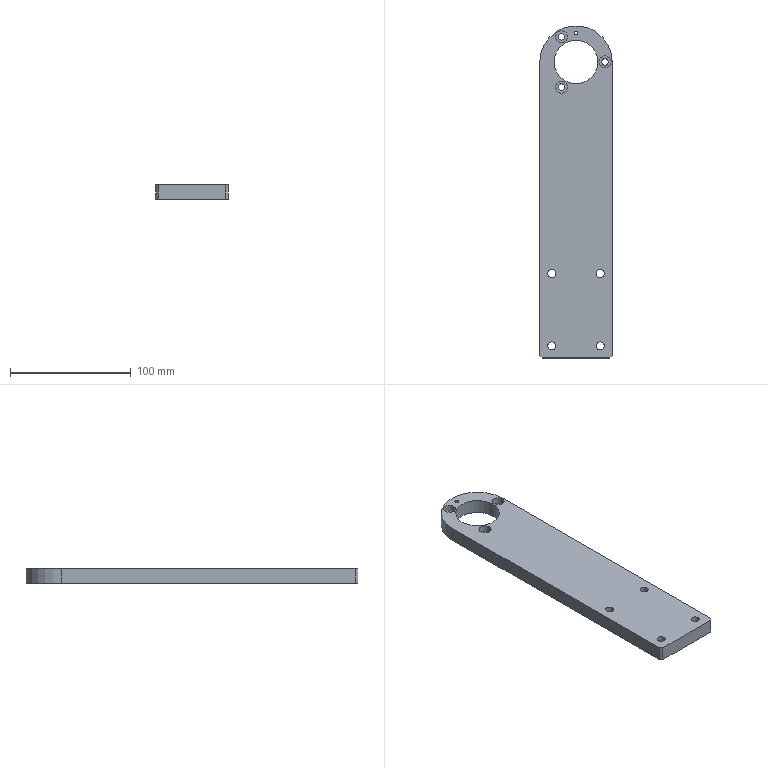Component | SolidWorks | JYTBJ-HeaderPlateSupportFrame-1 | 1 solid | 47 faces | box 60 x 275 x 12 mm | volume 175843 mm3 | cylinder 33 | plane 14 | commonest cylinder face diameters 11 x8 6.6 x8 10 x6 5.5 x6 3.3 x2 36.1 x2 60 x1
build123d program:
from build123d import *

# Parameters (mm, degrees)
SKETCH1_R                                            = 18.05
BOSS_EXTRUDE1_DEPTH                                  = 12
HOLE_SIZE_ACCORDING_TO_THE_TYPE_OF_HEXAG_D           = 5.5
HOLE_SIZE_ACCORDING_TO_THE_TYPE_OF_HEXAG_CBORE_D     = 10
HOLE_SIZE_ACCORDING_TO_THE_TYPE_OF_HEXAG_CBORE_DEPTH = 5.7
CIRPATTERN1_COUNT                                    = 3
HOLE_SIZE_ACCORDING_TO_THE_TYPE_OF_H_2_D             = 6.6
HOLE_SIZE_ACCORDING_TO_THE_TYPE_OF_H_2_CBORE_D       = 11
HOLE_SIZE_ACCORDING_TO_THE_TYPE_OF_H_2_CBORE_DEPTH   = 6.8
M4_TAPPED_HOLE1_D                                    = 3.3
CHAMFER1_SIZE                                        = 2


with BuildPart() as part:
    # Sketch1 → Boss-Extrude1 (new body)
    with BuildSketch(Plane.XY):
        with BuildLine():
            Line((-30, 0), (30, 0))
            Line((30, 0), (30, 245))
            ThreePointArc((30, 245), (0, 275), (-30, 245))
            Line((-30, 245), (-30, 0))
        make_face()
        with Locations((0, 245)):
            Circle(SKETCH1_R, mode=Mode.SUBTRACT)
    extrude(amount=BOSS_EXTRUDE1_DEPTH)

    # Hole Size according to the type of Hexag (through all)
    with Locations(Plane.XY.offset(12)):
        with Locations((24, 245)):
            hole_size_according_to_the_type_of_hexag = CounterBoreHole(HOLE_SIZE_ACCORDING_TO_THE_TYPE_OF_HEXAG_D / 2, HOLE_SIZE_ACCORDING_TO_THE_TYPE_OF_HEXAG_CBORE_D / 2, HOLE_SIZE_ACCORDING_TO_THE_TYPE_OF_HEXAG_CBORE_DEPTH)

    # CirPattern1: Hole Size according to the type of Hexag ×3 about axis
    cirpattern1_axis = Axis((0, 245, 0), (0, 0, 1))
    for i in range(1, CIRPATTERN1_COUNT):
        add(hole_size_according_to_the_type_of_hexag.rotate(cirpattern1_axis, i * 360 / CIRPATTERN1_COUNT), mode=Mode.SUBTRACT)

    # Hole Size according to the type of H 2 (through all)
    with Locations(Plane(origin=(0, 0, 0), x_dir=(-1, 0, 0), z_dir=(0, 0, -1))):
        with Locations((-20, 70), (-20, 10), (20, 70), (20, 10)):
            CounterBoreHole(HOLE_SIZE_ACCORDING_TO_THE_TYPE_OF_H_2_D / 2, HOLE_SIZE_ACCORDING_TO_THE_TYPE_OF_H_2_CBORE_D / 2, HOLE_SIZE_ACCORDING_TO_THE_TYPE_OF_H_2_CBORE_DEPTH)

    # M4 Tapped Hole1 (through all)
    with Locations(Plane.XY.offset(12)):
        with Locations((0, 269)):
            Hole(M4_TAPPED_HOLE1_D / 2)

    # Chamfer1
    chamfer1_edges = [part.edges().sort_by_distance(p)[0] for p in [
        (30, 0, 6),
        (-30, 0, 6),
    ]]
    chamfer(chamfer1_edges, length=CHAMFER1_SIZE)


solid = part.part

# Placed as in the assembly
solid = solid.moved(Location((3.373, -148.122, -6), (0, 0, 0)))